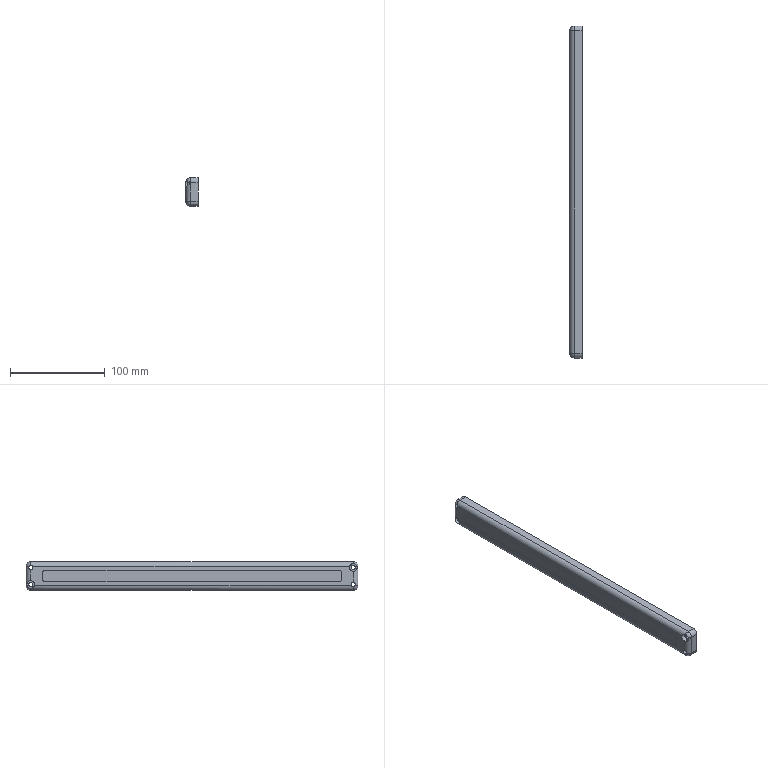Component | SolidWorks | A4-NA2-N16-L-1 | 1 solid | 41 faces | volume 127367 mm3 | cylinder 24 | plane 13 | sphere 4 | commonest cylinder face diameters 10 x8 4.6 x4 8.25 x4 4.3 x4 4 x4